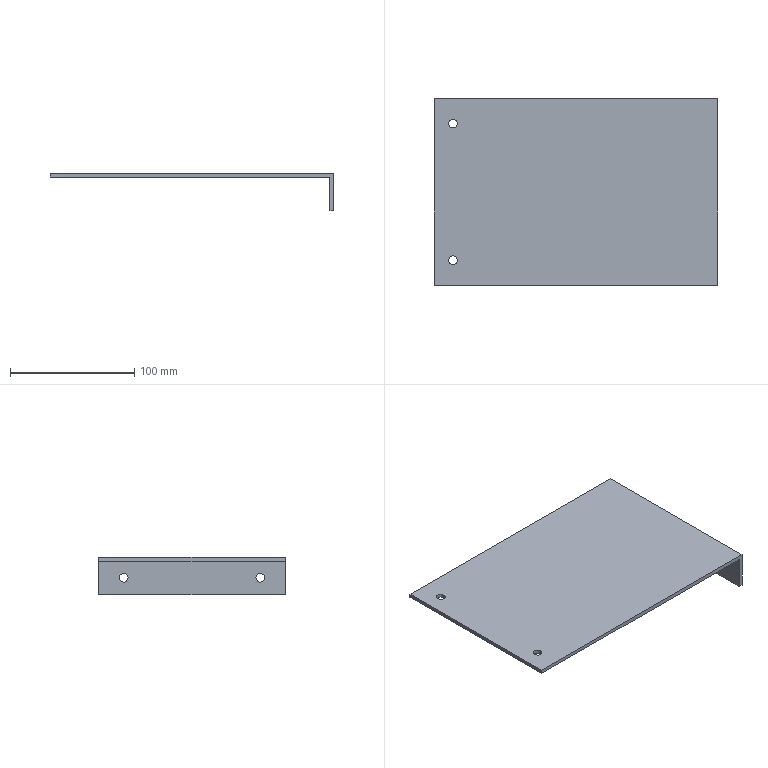Component | SolidWorks | LowerRightPlateBracket-1 | 1 solid | 16 faces | box 228 x 150 x 30 mm | volume 114288 mm3 | cylinder 8 | plane 8 | commonest cylinder face diameters 7 x8
build123d program:
from build123d import *

# Parameters (mm, degrees)
EXTRUDE_THIN1_DEPTH = 150
SKETCH3_R           = 3.5
CUT_EXTRUDE1_DEPTH  = 10
SKETCH4_R           = 3.5
CUT_EXTRUDE2_DEPTH  = 3


with BuildPart() as part:
    # Sketch2 → Extrude-Thin1 (new body)
    with BuildSketch(Plane.XY):
        Polygon((-68.157, 8.474), (-38.157, 8.474), (-38.157, -219.526), (-41.157, -219.526), (-41.157, 5.474), (-68.157, 5.474), align=None)
    extrude(amount=EXTRUDE_THIN1_DEPTH)

    # Sketch3 → Cut-Extrude1 (cut)
    with BuildSketch(Plane.ZY.offset(41.157)):
        with Locations(Location((20, -204.526, 0), (0, 0, 270))):
            Circle(SKETCH3_R)
        with Locations(Location((130, -204.526, 0), (0, 0, 270))):
            Circle(SKETCH3_R)
    extrude(amount=-CUT_EXTRUDE1_DEPTH, mode=Mode.SUBTRACT)

    # Sketch4 → Cut-Extrude2 (cut)
    with BuildSketch(Plane.XZ.offset(-5.474)):
        with Locations(Location((-54.657, 130, 0), (0, 0, 270))):
            Circle(SKETCH4_R)
        with Locations(Location((-54.657, 20, 0), (0, 0, 270))):
            Circle(SKETCH4_R)
    extrude(amount=-CUT_EXTRUDE2_DEPTH, mode=Mode.SUBTRACT)


solid = part.part

# Placed as in the assembly
solid = solid.moved(Location((754.977, -876.416, -330.362), (-90, 0, -90)))
STEP:
#1=CARTESIAN_POINT('',(30.057,-33.579,-15.158));
#2=VERTEX_POINT('',#1);
#3=CARTESIAN_POINT('',(30.057,-33.855,-15.158));
#4=VERTEX_POINT('',#3);
#5=CARTESIAN_POINT('',(30.057,-33.717,-15.158));
#6=DIRECTION('',(-1.,-0.,0.));
#7=DIRECTION('',(0.,-1.,0.));
#8=AXIS2_PLACEMENT_3D('',#5,#6,#7);
#9=CIRCLE('',#8,0.1378);
#10=EDGE_CURVE('',#2,#4,#9,.T.);
#11=ORIENTED_EDGE('',*,*,#10,.F.);
#12=CARTESIAN_POINT('',(29.939,-33.579,-15.158));
#13=VERTEX_POINT('',#12);
#14=CARTESIAN_POINT('',(30.057,-33.579,-15.158));
#15=DIRECTION('',(-1.,-0.,0.));
#16=VECTOR('',#15,39.37);
#17=LINE('',#14,#16);
#18=EDGE_CURVE('',#2,#13,#17,.T.);
#19=ORIENTED_EDGE('',*,*,#18,.T.);
#20=CARTESIAN_POINT('',(29.939,-33.855,-15.158));
#21=VERTEX_POINT('',#20);
#22=CARTESIAN_POINT('',(29.939,-33.717,-15.158));
#23=DIRECTION('',(-1.,-0.,0.));
#24=DIRECTION('',(0.,-1.,0.));
#25=AXIS2_PLACEMENT_3D('',#22,#23,#24);
#26=CIRCLE('',#25,0.1378);
#27=EDGE_CURVE('',#13,#21,#26,.T.);
#28=ORIENTED_EDGE('',*,*,#27,.T.);
#29=CARTESIAN_POINT('',(30.057,-33.855,-15.158));
#30=DIRECTION('',(-1.,-0.,0.));
#31=VECTOR('',#30,39.37);
#32=LINE('',#29,#31);
#33=EDGE_CURVE('',#4,#21,#32,.T.);
#34=ORIENTED_EDGE('',*,*,#33,.F.);
#35=EDGE_LOOP('',(#11,#19,#28,#34));
#36=FACE_OUTER_BOUND('',#35,.T.);
#37=CARTESIAN_POINT('',(30.057,-33.717,-15.158));
#38=DIRECTION('',(-1.,-0.,0.));
#39=DIRECTION('',(0.,-1.,0.));
#40=AXIS2_PLACEMENT_3D('',#37,#38,#39);
#41=CYLINDRICAL_SURFACE('',#40,0.1378);
#42=ADVANCED_FACE('',(#36),#41,.F.);
#43=CARTESIAN_POINT('',(30.057,-29.249,-15.158));
#44=VERTEX_POINT('',#43);
#45=CARTESIAN_POINT('',(30.057,-29.524,-15.158));
#46=VERTEX_POINT('',#45);
#47=CARTESIAN_POINT('',(30.057,-29.386,-15.158));
#48=DIRECTION('',(-1.,-0.,0.));
#49=DIRECTION('',(0.,-1.,0.));
#50=AXIS2_PLACEMENT_3D('',#47,#48,#49);
#51=CIRCLE('',#50,0.1378);
#52=EDGE_CURVE('',#44,#46,#51,.T.);
#53=ORIENTED_EDGE('',*,*,#52,.F.);
#54=CARTESIAN_POINT('',(29.939,-29.249,-15.158));
#55=VERTEX_POINT('',#54);
#56=CARTESIAN_POINT('',(30.057,-29.249,-15.158));
#57=DIRECTION('',(-1.,-0.,0.));
#58=VECTOR('',#57,39.37);
#59=LINE('',#56,#58);
#60=EDGE_CURVE('',#44,#55,#59,.T.);
#61=ORIENTED_EDGE('',*,*,#60,.T.);
#62=CARTESIAN_POINT('',(29.939,-29.524,-15.158));
#63=VERTEX_POINT('',#62);
#64=CARTESIAN_POINT('',(29.939,-29.386,-15.158));
#65=DIRECTION('',(-1.,-0.,0.));
#66=DIRECTION('',(0.,-1.,0.));
#67=AXIS2_PLACEMENT_3D('',#64,#65,#66);
#68=CIRCLE('',#67,0.1378);
#69=EDGE_CURVE('',#55,#63,#68,.T.);
#70=ORIENTED_EDGE('',*,*,#69,.T.);
#71=CARTESIAN_POINT('',(30.057,-29.524,-15.158));
#72=DIRECTION('',(-1.,-0.,0.));
#73=VECTOR('',#72,39.37);
#74=LINE('',#71,#73);
#75=EDGE_CURVE('',#46,#63,#74,.T.);
#76=ORIENTED_EDGE('',*,*,#75,.F.);
#77=EDGE_LOOP('',(#53,#61,#70,#76));
#78=FACE_OUTER_BOUND('',#77,.T.);
#79=CARTESIAN_POINT('',(30.057,-29.386,-15.158));
#80=DIRECTION('',(-1.,-0.,0.));
#81=DIRECTION('',(0.,-1.,0.));
#82=AXIS2_PLACEMENT_3D('',#79,#80,#81);
#83=CYLINDRICAL_SURFACE('',#82,0.1378);
#84=ADVANCED_FACE('',(#78),#83,.F.);
#85=CARTESIAN_POINT('',(21.533,-29.386,-14.509));
#86=VERTEX_POINT('',#85);
#87=CARTESIAN_POINT('',(21.809,-29.386,-14.509));
#88=VERTEX_POINT('',#87);
#89=CARTESIAN_POINT('',(21.671,-29.386,-14.509));
#90=DIRECTION('',(0.,-0.,1.));
#91=DIRECTION('',(1.,0.,0.));
#92=AXIS2_PLACEMENT_3D('',#89,#90,#91);
#93=CIRCLE('',#92,0.1378);
#94=EDGE_CURVE('',#86,#88,#93,.T.);
#95=ORIENTED_EDGE('',*,*,#94,.T.);
#96=CARTESIAN_POINT('',(21.809,-29.386,-14.627));
#97=VERTEX_POINT('',#96);
#98=CARTESIAN_POINT('',(21.809,-29.386,-14.233));
#99=DIRECTION('',(-0.,0.,-1.));
#100=VECTOR('',#99,39.37);
#101=LINE('',#98,#100);
#102=EDGE_CURVE('',#88,#97,#101,.T.);
#103=ORIENTED_EDGE('',*,*,#102,.T.);
#104=CARTESIAN_POINT('',(21.533,-29.386,-14.627));
#105=VERTEX_POINT('',#104);
#106=CARTESIAN_POINT('',(21.671,-29.386,-14.627));
#107=DIRECTION('',(-0.,0.,-1.));
#108=DIRECTION('',(-1.,0.,0.));
#109=AXIS2_PLACEMENT_3D('',#106,#107,#108);
#110=CIRCLE('',#109,0.1378);
#111=EDGE_CURVE('',#97,#105,#110,.T.);
#112=ORIENTED_EDGE('',*,*,#111,.T.);
#113=CARTESIAN_POINT('',(21.533,-29.386,-14.233));
#114=DIRECTION('',(-0.,0.,-1.));
#115=VECTOR('',#114,39.37);
#116=LINE('',#113,#115);
#117=EDGE_CURVE('',#86,#105,#116,.T.);
#118=ORIENTED_EDGE('',*,*,#117,.F.);
#119=EDGE_LOOP('',(#95,#103,#112,#118));
#120=FACE_OUTER_BOUND('',#119,.T.);
#121=CARTESIAN_POINT('',(21.671,-29.386,-14.233));
#122=DIRECTION('',(-0.,0.,-1.));
#123=DIRECTION('',(-1.,0.,0.));
#124=AXIS2_PLACEMENT_3D('',#121,#122,#123);
#125=CYLINDRICAL_SURFACE('',#124,0.1378);
#126=ADVANCED_FACE('',(#120),#125,.F.);
#127=CARTESIAN_POINT('',(21.533,-33.717,-14.509));
#128=VERTEX_POINT('',#127);
#129=CARTESIAN_POINT('',(21.809,-33.717,-14.509));
#130=VERTEX_POINT('',#129);
#131=CARTESIAN_POINT('',(21.671,-33.717,-14.509));
#132=DIRECTION('',(0.,-0.,1.));
#133=DIRECTION('',(1.,0.,0.));
#134=AXIS2_PLACEMENT_3D('',#131,#132,#133);
#135=CIRCLE('',#134,0.1378);
#136=EDGE_CURVE('',#128,#130,#135,.T.);
#137=ORIENTED_EDGE('',*,*,#136,.T.);
#138=CARTESIAN_POINT('',(21.809,-33.717,-14.627));
#139=VERTEX_POINT('',#138);
#140=CARTESIAN_POINT('',(21.809,-33.717,-14.233));
#141=DIRECTION('',(-0.,0.,-1.));
#142=VECTOR('',#141,39.37);
#143=LINE('',#140,#142);
#144=EDGE_CURVE('',#130,#139,#143,.T.);
#145=ORIENTED_EDGE('',*,*,#144,.T.);
#146=CARTESIAN_POINT('',(21.533,-33.717,-14.627));
#147=VERTEX_POINT('',#146);
#148=CARTESIAN_POINT('',(21.671,-33.717,-14.627));
#149=DIRECTION('',(-0.,0.,-1.));
#150=DIRECTION('',(-1.,0.,0.));
#151=AXIS2_PLACEMENT_3D('',#148,#149,#150);
#152=CIRCLE('',#151,0.1378);
#153=EDGE_CURVE('',#139,#147,#152,.T.);
#154=ORIENTED_EDGE('',*,*,#153,.T.);
#155=CARTESIAN_POINT('',(21.533,-33.717,-14.233));
#156=DIRECTION('',(-0.,0.,-1.));
#157=VECTOR('',#156,39.37);
#158=LINE('',#155,#157);
#159=EDGE_CURVE('',#128,#147,#158,.T.);
#160=ORIENTED_EDGE('',*,*,#159,.F.);
#161=EDGE_LOOP('',(#137,#145,#154,#160));
#162=FACE_OUTER_BOUND('',#161,.T.);
#163=CARTESIAN_POINT('',(21.671,-33.717,-14.233));
#164=DIRECTION('',(-0.,0.,-1.));
#165=DIRECTION('',(-1.,0.,0.));
#166=AXIS2_PLACEMENT_3D('',#163,#164,#165);
#167=CYLINDRICAL_SURFACE('',#166,0.1378);
#168=ADVANCED_FACE('',(#162),#167,.F.);
#169=CARTESIAN_POINT('',(21.671,-29.386,-14.627));
#170=DIRECTION('',(-0.,0.,-1.));
#171=DIRECTION('',(-1.,0.,0.));
#172=AXIS2_PLACEMENT_3D('',#169,#170,#171);
#173=CIRCLE('',#172,0.1378);
#174=EDGE_CURVE('',#105,#97,#173,.T.);
#175=ORIENTED_EDGE('',*,*,#174,.F.);
#176=ORIENTED_EDGE('',*,*,#111,.F.);
#177=EDGE_LOOP('',(#175,#176));
#178=FACE_BOUND('',#177,.T.);
#179=CARTESIAN_POINT('',(21.671,-33.717,-14.627));
#180=DIRECTION('',(-0.,0.,-1.));
#181=DIRECTION('',(-1.,0.,0.));
#182=AXIS2_PLACEMENT_3D('',#179,#180,#181);
#183=CIRCLE('',#182,0.1378);
#184=EDGE_CURVE('',#147,#139,#183,.T.);
#185=ORIENTED_EDGE('',*,*,#184,.F.);
#186=ORIENTED_EDGE('',*,*,#153,.F.);
#187=EDGE_LOOP('',(#185,#186));
#188=FACE_BOUND('',#187,.T.);
#189=CARTESIAN_POINT('',(29.939,-34.505,-14.627));
#190=VERTEX_POINT('',#189);
#191=CARTESIAN_POINT('',(21.081,-34.505,-14.627));
#192=VERTEX_POINT('',#191);
#193=CARTESIAN_POINT('',(30.057,-34.505,-14.627));
#194=DIRECTION('',(-1.,-0.,0.));
#195=VECTOR('',#194,39.37);
#196=LINE('',#193,#195);
#197=EDGE_CURVE('',#190,#192,#196,.T.);
#198=ORIENTED_EDGE('',*,*,#197,.T.);
#199=CARTESIAN_POINT('',(21.081,-28.599,-14.627));
#200=VERTEX_POINT('',#199);
#201=CARTESIAN_POINT('',(21.081,-28.599,-14.627));
#202=DIRECTION('',(0.,-1.,-0.));
#203=VECTOR('',#202,39.37);
#204=LINE('',#201,#203);
#205=EDGE_CURVE('',#200,#192,#204,.T.);
#206=ORIENTED_EDGE('',*,*,#205,.F.);
#207=CARTESIAN_POINT('',(29.939,-28.599,-14.627));
#208=VERTEX_POINT('',#207);
#209=CARTESIAN_POINT('',(30.057,-28.599,-14.627));
#210=DIRECTION('',(-1.,-0.,0.));
#211=VECTOR('',#210,39.37);
#212=LINE('',#209,#211);
#213=EDGE_CURVE('',#208,#200,#212,.T.);
#214=ORIENTED_EDGE('',*,*,#213,.F.);
#215=CARTESIAN_POINT('',(29.939,-28.599,-14.627));
#216=DIRECTION('',(0.,-1.,-0.));
#217=VECTOR('',#216,39.37);
#218=LINE('',#215,#217);
#219=EDGE_CURVE('',#208,#190,#218,.T.);
#220=ORIENTED_EDGE('',*,*,#219,.T.);
#221=EDGE_LOOP('',(#198,#206,#214,#220));
#222=FACE_OUTER_BOUND('',#221,.T.);
#223=CARTESIAN_POINT('',(30.057,-28.599,-14.627));
#224=DIRECTION('',(0.,-0.,1.));
#225=DIRECTION('',(1.,0.,-0.));
#226=AXIS2_PLACEMENT_3D('',#223,#224,#225);
#227=PLANE('',#226);
#228=ADVANCED_FACE('',(#178,#188,#222),#227,.F.);
#229=CARTESIAN_POINT('',(21.081,-34.505,-14.509));
#230=VERTEX_POINT('',#229);
#231=CARTESIAN_POINT('',(21.081,-34.505,-14.509));
#232=DIRECTION('',(0.,0.,-1.));
#233=VECTOR('',#232,39.37);
#234=LINE('',#231,#233);
#235=EDGE_CURVE('',#230,#192,#234,.T.);
#236=ORIENTED_EDGE('',*,*,#235,.F.);
#237=CARTESIAN_POINT('',(21.081,-28.599,-14.509));
#238=VERTEX_POINT('',#237);
#239=CARTESIAN_POINT('',(21.081,-28.599,-14.509));
#240=DIRECTION('',(0.,-1.,-0.));
#241=VECTOR('',#240,39.37);
#242=LINE('',#239,#241);
#243=EDGE_CURVE('',#238,#230,#242,.T.);
#244=ORIENTED_EDGE('',*,*,#243,.F.);
#245=CARTESIAN_POINT('',(21.081,-28.599,-14.509));
#246=DIRECTION('',(0.,0.,-1.));
#247=VECTOR('',#246,39.37);
#248=LINE('',#245,#247);
#249=EDGE_CURVE('',#238,#200,#248,.T.);
#250=ORIENTED_EDGE('',*,*,#249,.T.);
#251=ORIENTED_EDGE('',*,*,#205,.T.);
#252=EDGE_LOOP('',(#236,#244,#250,#251));
#253=FACE_OUTER_BOUND('',#252,.T.);
#254=CARTESIAN_POINT('',(21.081,-28.599,-14.509));
#255=DIRECTION('',(-1.,-0.,0.));
#256=DIRECTION('',(0.,-1.,-0.));
#257=AXIS2_PLACEMENT_3D('',#254,#255,#256);
#258=PLANE('',#257);
#259=ADVANCED_FACE('',(#253),#258,.T.);
#260=ORIENTED_EDGE('',*,*,#94,.F.);
#261=CARTESIAN_POINT('',(21.671,-29.386,-14.509));
#262=DIRECTION('',(0.,-0.,1.));
#263=DIRECTION('',(1.,0.,0.));
#264=AXIS2_PLACEMENT_3D('',#261,#262,#263);
#265=CIRCLE('',#264,0.1378);
#266=EDGE_CURVE('',#88,#86,#265,.T.);
#267=ORIENTED_EDGE('',*,*,#266,.F.);
#268=EDGE_LOOP('',(#260,#267));
#269=FACE_BOUND('',#268,.T.);
#270=ORIENTED_EDGE('',*,*,#136,.F.);
#271=CARTESIAN_POINT('',(21.671,-33.717,-14.509));
#272=DIRECTION('',(0.,-0.,1.));
#273=DIRECTION('',(1.,0.,0.));
#274=AXIS2_PLACEMENT_3D('',#271,#272,#273);
#275=CIRCLE('',#274,0.1378);
#276=EDGE_CURVE('',#130,#128,#275,.T.);
#277=ORIENTED_EDGE('',*,*,#276,.F.);
#278=EDGE_LOOP('',(#270,#277));
#279=FACE_BOUND('',#278,.T.);
#280=CARTESIAN_POINT('',(30.057,-34.505,-14.509));
#281=VERTEX_POINT('',#280);
#282=CARTESIAN_POINT('',(30.057,-34.505,-14.509));
#283=DIRECTION('',(-1.,-0.,0.));
#284=VECTOR('',#283,39.37);
#285=LINE('',#282,#284);
#286=EDGE_CURVE('',#281,#230,#285,.T.);
#287=ORIENTED_EDGE('',*,*,#286,.F.);
#288=CARTESIAN_POINT('',(30.057,-28.599,-14.509));
#289=VERTEX_POINT('',#288);
#290=CARTESIAN_POINT('',(30.057,-28.599,-14.509));
#291=DIRECTION('',(0.,-1.,-0.));
#292=VECTOR('',#291,39.37);
#293=LINE('',#290,#292);
#294=EDGE_CURVE('',#289,#281,#293,.T.);
#295=ORIENTED_EDGE('',*,*,#294,.F.);
#296=CARTESIAN_POINT('',(30.057,-28.599,-14.509));
#297=DIRECTION('',(-1.,-0.,0.));
#298=VECTOR('',#297,39.37);
#299=LINE('',#296,#298);
#300=EDGE_CURVE('',#289,#238,#299,.T.);
#301=ORIENTED_EDGE('',*,*,#300,.T.);
#302=ORIENTED_EDGE('',*,*,#243,.T.);
#303=EDGE_LOOP('',(#287,#295,#301,#302));
#304=FACE_OUTER_BOUND('',#303,.T.);
#305=CARTESIAN_POINT('',(30.057,-28.599,-14.509));
#306=DIRECTION('',(0.,-0.,1.));
#307=DIRECTION('',(1.,0.,-0.));
#308=AXIS2_PLACEMENT_3D('',#305,#306,#307);
#309=PLANE('',#308);
#310=ADVANCED_FACE('',(#269,#279,#304),#309,.T.);
#311=CARTESIAN_POINT('',(30.057,-33.717,-15.158));
#312=DIRECTION('',(-1.,-0.,0.));
#313=DIRECTION('',(0.,-1.,0.));
#314=AXIS2_PLACEMENT_3D('',#311,#312,#313);
#315=CIRCLE('',#314,0.1378);
#316=EDGE_CURVE('',#4,#2,#315,.T.);
#317=ORIENTED_EDGE('',*,*,#316,.T.);
#318=ORIENTED_EDGE('',*,*,#10,.T.);
#319=EDGE_LOOP('',(#317,#318));
#320=FACE_BOUND('',#319,.T.);
#321=CARTESIAN_POINT('',(30.057,-29.386,-15.158));
#322=DIRECTION('',(-1.,-0.,0.));
#323=DIRECTION('',(0.,-1.,0.));
#324=AXIS2_PLACEMENT_3D('',#321,#322,#323);
#325=CIRCLE('',#324,0.1378);
#326=EDGE_CURVE('',#46,#44,#325,.T.);
#327=ORIENTED_EDGE('',*,*,#326,.T.);
#328=ORIENTED_EDGE('',*,*,#52,.T.);
#329=EDGE_LOOP('',(#327,#328));
#330=FACE_BOUND('',#329,.T.);
#331=CARTESIAN_POINT('',(30.057,-34.505,-15.69));
#332=VERTEX_POINT('',#331);
#333=CARTESIAN_POINT('',(30.057,-34.505,-15.69));
#334=DIRECTION('',(-0.,-0.,1.));
#335=VECTOR('',#334,39.37);
#336=LINE('',#333,#335);
#337=EDGE_CURVE('',#332,#281,#336,.T.);
#338=ORIENTED_EDGE('',*,*,#337,.F.);
#339=CARTESIAN_POINT('',(30.057,-28.599,-15.69));
#340=VERTEX_POINT('',#339);
#341=CARTESIAN_POINT('',(30.057,-28.599,-15.69));
#342=DIRECTION('',(0.,-1.,-0.));
#343=VECTOR('',#342,39.37);
#344=LINE('',#341,#343);
#345=EDGE_CURVE('',#340,#332,#344,.T.);
#346=ORIENTED_EDGE('',*,*,#345,.F.);
#347=CARTESIAN_POINT('',(30.057,-28.599,-15.69));
#348=DIRECTION('',(-0.,-0.,1.));
#349=VECTOR('',#348,39.37);
#350=LINE('',#347,#349);
#351=EDGE_CURVE('',#340,#289,#350,.T.);
#352=ORIENTED_EDGE('',*,*,#351,.T.);
#353=ORIENTED_EDGE('',*,*,#294,.T.);
#354=EDGE_LOOP('',(#338,#346,#352,#353));
#355=FACE_OUTER_BOUND('',#354,.T.);
#356=CARTESIAN_POINT('',(30.057,-28.599,-15.69));
#357=DIRECTION('',(1.,0.,-0.));
#358=DIRECTION('',(-0.,1.,0.));
#359=AXIS2_PLACEMENT_3D('',#356,#357,#358);
#360=PLANE('',#359);
#361=ADVANCED_FACE('',(#320,#330,#355),#360,.T.);
#362=CARTESIAN_POINT('',(29.939,-34.505,-15.69));
#363=VERTEX_POINT('',#362);
#364=CARTESIAN_POINT('',(29.939,-34.505,-15.69));
#365=DIRECTION('',(1.,0.,-0.));
#366=VECTOR('',#365,39.37);
#367=LINE('',#364,#366);
#368=EDGE_CURVE('',#363,#332,#367,.T.);
#369=ORIENTED_EDGE('',*,*,#368,.F.);
#370=CARTESIAN_POINT('',(29.939,-28.599,-15.69));
#371=VERTEX_POINT('',#370);
#372=CARTESIAN_POINT('',(29.939,-28.599,-15.69));
#373=DIRECTION('',(0.,-1.,-0.));
#374=VECTOR('',#373,39.37);
#375=LINE('',#372,#374);
#376=EDGE_CURVE('',#371,#363,#375,.T.);
#377=ORIENTED_EDGE('',*,*,#376,.F.);
#378=CARTESIAN_POINT('',(29.939,-28.599,-15.69));
#379=DIRECTION('',(1.,0.,-0.));
#380=VECTOR('',#379,39.37);
#381=LINE('',#378,#380);
#382=EDGE_CURVE('',#371,#340,#381,.T.);
#383=ORIENTED_EDGE('',*,*,#382,.T.);
#384=ORIENTED_EDGE('',*,*,#345,.T.);
#385=EDGE_LOOP('',(#369,#377,#383,#384));
#386=FACE_OUTER_BOUND('',#385,.T.);
#387=CARTESIAN_POINT('',(29.939,-28.599,-15.69));
#388=DIRECTION('',(0.,0.,-1.));
#389=DIRECTION('',(-0.,1.,0.));
#390=AXIS2_PLACEMENT_3D('',#387,#388,#389);
#391=PLANE('',#390);
#392=ADVANCED_FACE('',(#386),#391,.T.);
#393=CARTESIAN_POINT('',(29.939,-33.717,-15.158));
#394=DIRECTION('',(-1.,-0.,0.));
#395=DIRECTION('',(0.,-1.,0.));
#396=AXIS2_PLACEMENT_3D('',#393,#394,#395);
#397=CIRCLE('',#396,0.1378);
#398=EDGE_CURVE('',#21,#13,#397,.T.);
#399=ORIENTED_EDGE('',*,*,#398,.F.);
#400=ORIENTED_EDGE('',*,*,#27,.F.);
#401=EDGE_LOOP('',(#399,#400));
#402=FACE_BOUND('',#401,.T.);
#403=CARTESIAN_POINT('',(29.939,-29.386,-15.158));
#404=DIRECTION('',(-1.,-0.,0.));
#405=DIRECTION('',(0.,-1.,0.));
#406=AXIS2_PLACEMENT_3D('',#403,#404,#405);
#407=CIRCLE('',#406,0.1378);
#408=EDGE_CURVE('',#63,#55,#407,.T.);
#409=ORIENTED_EDGE('',*,*,#408,.F.);
#410=ORIENTED_EDGE('',*,*,#69,.F.);
#411=EDGE_LOOP('',(#409,#410));
#412=FACE_BOUND('',#411,.T.);
#413=CARTESIAN_POINT('',(29.939,-34.505,-15.69));
#414=DIRECTION('',(-0.,-0.,1.));
#415=VECTOR('',#414,39.37);
#416=LINE('',#413,#415);
#417=EDGE_CURVE('',#363,#190,#416,.T.);
#418=ORIENTED_EDGE('',*,*,#417,.T.);
#419=ORIENTED_EDGE('',*,*,#219,.F.);
#420=CARTESIAN_POINT('',(29.939,-28.599,-15.69));
#421=DIRECTION('',(-0.,-0.,1.));
#422=VECTOR('',#421,39.37);
#423=LINE('',#420,#422);
#424=EDGE_CURVE('',#371,#208,#423,.T.);
#425=ORIENTED_EDGE('',*,*,#424,.F.);
#426=ORIENTED_EDGE('',*,*,#376,.T.);
#427=EDGE_LOOP('',(#418,#419,#425,#426));
#428=FACE_OUTER_BOUND('',#427,.T.);
#429=CARTESIAN_POINT('',(29.939,-28.599,-15.69));
#430=DIRECTION('',(1.,0.,-0.));
#431=DIRECTION('',(-0.,1.,0.));
#432=AXIS2_PLACEMENT_3D('',#429,#430,#431);
#433=PLANE('',#432);
#434=ADVANCED_FACE('',(#402,#412,#428),#433,.F.);
#435=ORIENTED_EDGE('',*,*,#213,.T.);
#436=ORIENTED_EDGE('',*,*,#249,.F.);
#437=ORIENTED_EDGE('',*,*,#300,.F.);
#438=ORIENTED_EDGE('',*,*,#351,.F.);
#439=ORIENTED_EDGE('',*,*,#382,.F.);
#440=ORIENTED_EDGE('',*,*,#424,.T.);
#441=EDGE_LOOP('',(#435,#436,#437,#438,#439,#440));
#442=FACE_OUTER_BOUND('',#441,.T.);
#443=CARTESIAN_POINT('',(29.723,-28.599,-13.006));
#444=DIRECTION('',(0.,-1.,-0.));
#445=DIRECTION('',(0.,0.,-1.));
#446=AXIS2_PLACEMENT_3D('',#443,#444,#445);
#447=PLANE('',#446);
#448=ADVANCED_FACE('',(#442),#447,.F.);
#449=ORIENTED_EDGE('',*,*,#197,.F.);
#450=ORIENTED_EDGE('',*,*,#417,.F.);
#451=ORIENTED_EDGE('',*,*,#368,.T.);
#452=ORIENTED_EDGE('',*,*,#337,.T.);
#453=ORIENTED_EDGE('',*,*,#286,.T.);
#454=ORIENTED_EDGE('',*,*,#235,.T.);
#455=EDGE_LOOP('',(#449,#450,#451,#452,#453,#454));
#456=FACE_OUTER_BOUND('',#455,.T.);
#457=CARTESIAN_POINT('',(29.723,-34.505,-13.006));
#458=DIRECTION('',(0.,-1.,-0.));
#459=DIRECTION('',(0.,0.,-1.));
#460=AXIS2_PLACEMENT_3D('',#457,#458,#459);
#461=PLANE('',#460);
#462=ADVANCED_FACE('',(#456),#461,.T.);
#463=ORIENTED_EDGE('',*,*,#144,.F.);
#464=ORIENTED_EDGE('',*,*,#276,.T.);
#465=ORIENTED_EDGE('',*,*,#159,.T.);
#466=ORIENTED_EDGE('',*,*,#184,.T.);
#467=EDGE_LOOP('',(#463,#464,#465,#466));
#468=FACE_OUTER_BOUND('',#467,.T.);
#469=CARTESIAN_POINT('',(21.671,-33.717,-14.233));
#470=DIRECTION('',(-0.,0.,-1.));
#471=DIRECTION('',(-1.,0.,0.));
#472=AXIS2_PLACEMENT_3D('',#469,#470,#471);
#473=CYLINDRICAL_SURFACE('',#472,0.1378);
#474=ADVANCED_FACE('',(#468),#473,.F.);
#475=ORIENTED_EDGE('',*,*,#102,.F.);
#476=ORIENTED_EDGE('',*,*,#266,.T.);
#477=ORIENTED_EDGE('',*,*,#117,.T.);
#478=ORIENTED_EDGE('',*,*,#174,.T.);
#479=EDGE_LOOP('',(#475,#476,#477,#478));
#480=FACE_OUTER_BOUND('',#479,.T.);
#481=CARTESIAN_POINT('',(21.671,-29.386,-14.233));
#482=DIRECTION('',(-0.,0.,-1.));
#483=DIRECTION('',(-1.,0.,0.));
#484=AXIS2_PLACEMENT_3D('',#481,#482,#483);
#485=CYLINDRICAL_SURFACE('',#484,0.1378);
#486=ADVANCED_FACE('',(#480),#485,.F.);
#487=ORIENTED_EDGE('',*,*,#60,.F.);
#488=ORIENTED_EDGE('',*,*,#326,.F.);
#489=ORIENTED_EDGE('',*,*,#75,.T.);
#490=ORIENTED_EDGE('',*,*,#408,.T.);
#491=EDGE_LOOP('',(#487,#488,#489,#490));
#492=FACE_OUTER_BOUND('',#491,.T.);
#493=CARTESIAN_POINT('',(30.057,-29.386,-15.158));
#494=DIRECTION('',(-1.,-0.,0.));
#495=DIRECTION('',(0.,-1.,0.));
#496=AXIS2_PLACEMENT_3D('',#493,#494,#495);
#497=CYLINDRICAL_SURFACE('',#496,0.1378);
#498=ADVANCED_FACE('',(#492),#497,.F.);
#499=ORIENTED_EDGE('',*,*,#18,.F.);
#500=ORIENTED_EDGE('',*,*,#316,.F.);
#501=ORIENTED_EDGE('',*,*,#33,.T.);
#502=ORIENTED_EDGE('',*,*,#398,.T.);
#503=EDGE_LOOP('',(#499,#500,#501,#502));
#504=FACE_OUTER_BOUND('',#503,.T.);
#505=CARTESIAN_POINT('',(30.057,-33.717,-15.158));
#506=DIRECTION('',(-1.,-0.,0.));
#507=DIRECTION('',(0.,-1.,0.));
#508=AXIS2_PLACEMENT_3D('',#505,#506,#507);
#509=CYLINDRICAL_SURFACE('',#508,0.1378);
#510=ADVANCED_FACE('',(#504),#509,.F.);
#511=CLOSED_SHELL('',(#42,#84,#126,#168,#228,#259,#310,#361,#392,#434,#448,#462,#474,#486,#498,#510));
#512=MANIFOLD_SOLID_BREP('',#511);
#513=CARTESIAN_POINT('',(0.,0.,0.));
#514=DIRECTION('',(0.,0.,1.));
#515=DIRECTION('',(1.,0.,0.));
#516=AXIS2_PLACEMENT_3D('',#513,#514,#515);
#517=(LENGTH_UNIT()NAMED_UNIT(*)SI_UNIT($,.METRE.));
#518=LENGTH_MEASURE_WITH_UNIT(LENGTH_MEASURE(0.0254),#517);
#519=DIMENSIONAL_EXPONENTS(1.,0.,0.,0.,0.,0.,0.);
#520=(CONVERSION_BASED_UNIT('',#518)LENGTH_UNIT()NAMED_UNIT(#519));
#521=UNCERTAINTY_MEASURE_WITH_UNIT(LENGTH_MEASURE(0.00001),#520,'','');
#522=(NAMED_UNIT(*)PLANE_ANGLE_UNIT()SI_UNIT($,.RADIAN.));
#523=(NAMED_UNIT(*)SI_UNIT($,.STERADIAN.)SOLID_ANGLE_UNIT());
#524=(GEOMETRIC_REPRESENTATION_CONTEXT(3)GLOBAL_UNCERTAINTY_ASSIGNED_CONTEXT((#521))GLOBAL_UNIT_ASSIGNED_CONTEXT((#520,#522,#523))REPRESENTATION_CONTEXT('',''));
#525=ADVANCED_BREP_SHAPE_REPRESENTATION('',(#512,#516),#524);
#526=COLOUR_RGB('',0.7922,0.8196,0.9333);
#527=FILL_AREA_STYLE_COLOUR('',#526);
#528=FILL_AREA_STYLE('',(#527));
#529=SURFACE_STYLE_FILL_AREA(#528);
#530=SURFACE_SIDE_STYLE('',(#529));
#531=SURFACE_STYLE_USAGE(.BOTH.,#530);
#532=PRESENTATION_STYLE_ASSIGNMENT((#531));
#533=STYLED_ITEM('',(#532),#512);
#534=PRESENTATION_LAYER_ASSIGNMENT('','',(#533));
#535=(LENGTH_UNIT()NAMED_UNIT(*)SI_UNIT($,.METRE.));
#536=LENGTH_MEASURE_WITH_UNIT(LENGTH_MEASURE(0.0254),#535);
#537=DIMENSIONAL_EXPONENTS(1.,0.,0.,0.,0.,0.,0.);
#538=(CONVERSION_BASED_UNIT('',#536)LENGTH_UNIT()NAMED_UNIT(#537));
#539=UNCERTAINTY_MEASURE_WITH_UNIT(LENGTH_MEASURE(0.00001),#538,'','');
#540=(NAMED_UNIT(*)PLANE_ANGLE_UNIT()SI_UNIT($,.RADIAN.));
#541=(NAMED_UNIT(*)SI_UNIT($,.STERADIAN.)SOLID_ANGLE_UNIT());
#542=(GEOMETRIC_REPRESENTATION_CONTEXT(3)GLOBAL_UNCERTAINTY_ASSIGNED_CONTEXT((#539))GLOBAL_UNIT_ASSIGNED_CONTEXT((#538,#540,#541))REPRESENTATION_CONTEXT('',''));
#543=MECHANICAL_DESIGN_GEOMETRIC_PRESENTATION_REPRESENTATION('',(#533),#542);